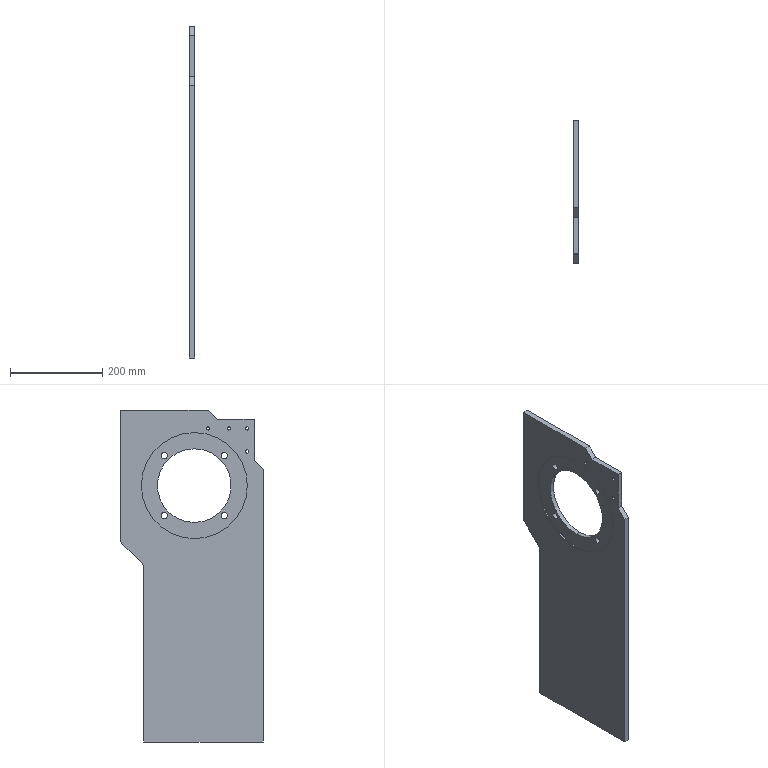Component | SolidWorks | JHK-A1002DriveWheelSupportPlateLeft-2 | 1 solid | 35 faces | box 12 x 310 x 720 mm | volume 2090542 mm3 | cylinder 22 | plane 13 | commonest cylinder face diameters 14 x8 6.8 x8 230 x2 160 x2 20 x2 | material Q235A
build123d program:
from build123d import *

# Parameters (mm, degrees)
BOSS_EXTRUDE1_DEPTH = 6
SKETCH2_R           = 80
CUT_EXTRUDE1_DEPTH  = 397.729
M8_TAPPED_HOLE1_D   = 6.8
SKETCH5_R           = 115
CUT_EXTRUDE2_DEPTH  = 2
M16_TAPPED_HOLE1_D  = 14
FILLET1_R           = 10


with BuildPart() as part:
    # Sketch1 → Boss-Extrude1 (new, symmetric)
    with BuildSketch(Plane(origin=(0, 0, 0), x_dir=(0, 0, -1), z_dir=(1, 0, 0))):
        Polygon((-355, 155), (-69, 155), (-19, 105), (365, 105), (365, -155), (-225, -155), (-245, -135), (-335, -135), (-335, -55), (-355, -35), align=None)
    extrude(amount=BOSS_EXTRUDE1_DEPTH, both=True)

    # Sketch2 → Cut-Extrude1 (cut, through all)
    with BuildSketch(Plane(origin=(6, 0, 0), x_dir=(0, 0, -1), z_dir=(1, 0, 0))):
        with Locations((-191, -5)):
            Circle(SKETCH2_R)
    extrude(amount=-CUT_EXTRUDE1_DEPTH, mode=Mode.SUBTRACT)

    # M8 Tapped Hole1 (through all)
    with Locations(Plane(origin=(6, 0, 0), x_dir=(0, 0, -1), z_dir=(1, 0, 0))):
        with Locations((-315, -120), (-265, -120), (-315, -80), (-315, -35)):
            Hole(M8_TAPPED_HOLE1_D / 2)

    # Sketch5 → Cut-Extrude2 (cut)
    with BuildSketch(Plane.ZY.offset(6)):
        with Locations((191, -5)):
            Circle(SKETCH5_R)
    extrude(amount=-CUT_EXTRUDE2_DEPTH, mode=Mode.SUBTRACT)

    # M16 Tapped Hole1 (through all)
    with Locations(Plane.ZY.offset(4)):
        with Locations((125.946, 60.054), (256.054, 60.054), (256.054, -70.054), (125.946, -70.054)):
            Hole(M16_TAPPED_HOLE1_D / 2)

    # Fillet1
    fillet1_edges = [part.edges().sort_by_distance(p)[0] for p in [
        (0, 155, 69),
        (0, 105, 19),
    ]]
    fillet(fillet1_edges, radius=FILLET1_R)


solid = part.part

# Placed as in the assembly
solid = solid.moved(Location((-79, 0, 0), (0, 0, 0)))